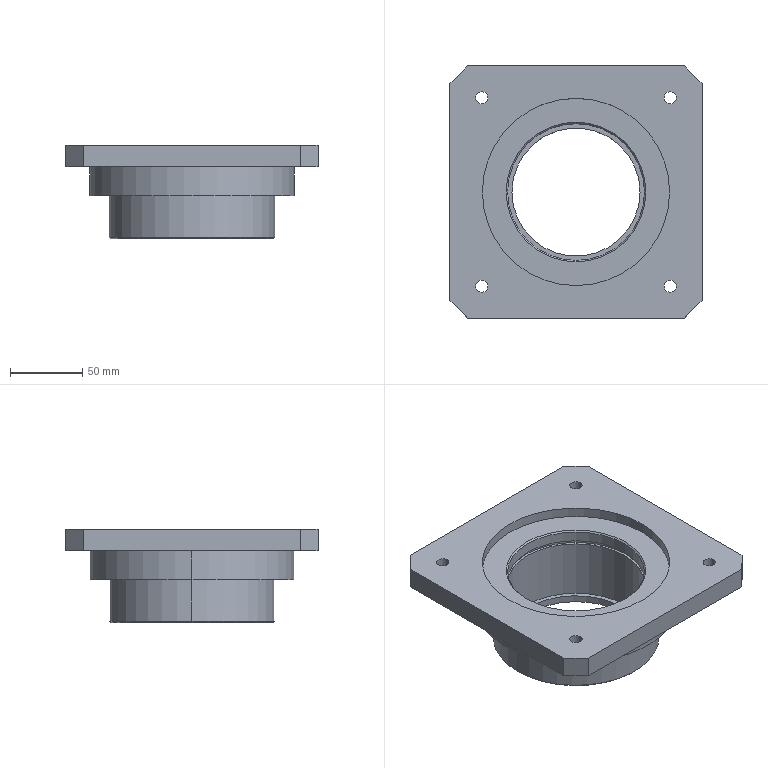Component | SolidWorks | PlanetaryReducer-PLF142BearingHousing-1 | 1 solid | 42 faces | box 175 x 175 x 65 mm | volume 578532 mm3 | cylinder 22 | plane 16 | cone 4 | commonest cylinder face diameters 8.5 x8 95 x4 130 x2 98.5 x2 142 x2 115 x2 89 x2
build123d program:
from build123d import *

# Parameters (mm, degrees)
SKETCH1_R           = 57.5
BOSS_EXTRUDE1_DEPTH = 30
SKETCH2_R           = 71
BOSS_EXTRUDE2_DEPTH = 20
SKETCH3_R           = 65
BOSS_EXTRUDE3_DEPTH = 8
SKETCH4_R           = 44.5
CUT_EXTRUDE1_DEPTH  = 116.957
SKETCH5_R           = 47.5
CUT_EXTRUDE2_DEPTH  = 53
CUT_EXTRUDE3_START  = -8.3
SKETCH6_R           = 49.25
CUT_EXTRUDE3_DEPTH  = 2.7
CHAMFER1_SIZE       = 1
SKETCH7_W           = 175
SKETCH7_H           = 175
SKETCH7_R           = 65
BOSS_EXTRUDE4_DEPTH = 15
CHAMFER2_SIZE       = 12
M10_TAPPED_HOLE1_D  = 8.5


with BuildPart() as part:
    # Sketch1 → Boss-Extrude1 (new body)
    with BuildSketch(Plane(origin=(0, 0, 0), x_dir=(1, 0, 0), z_dir=(0, 1, 0))):
        with Locations(Location((0, 0, 0), (0, 0, 270))):
            Circle(SKETCH1_R)
    extrude(amount=BOSS_EXTRUDE1_DEPTH)

    # Sketch2 → Boss-Extrude2 (add)
    with BuildSketch(Plane(origin=(0, 30, 0), x_dir=(1, 0, 0), z_dir=(0, 1, 0))):
        with Locations(Location((0, 0, 0), (0, 0, 270))):
            Circle(SKETCH2_R)
    extrude(amount=BOSS_EXTRUDE2_DEPTH)

    # Sketch3 → Boss-Extrude3 (add)
    with BuildSketch(Plane(origin=(0, 50, 0), x_dir=(1, 0, 0), z_dir=(0, 1, 0))):
        with Locations(Location((0, 0, 0), (0, 0, 270))):
            Circle(SKETCH3_R)
    extrude(amount=BOSS_EXTRUDE3_DEPTH)

    # Sketch4 → Cut-Extrude1 (cut, through all)
    with BuildSketch(Plane(origin=(0, 58, 0), x_dir=(1, 0, 0), z_dir=(0, 1, 0))):
        with Locations(Location((0, 0, 0), (0, 0, 270))):
            Circle(SKETCH4_R)
    extrude(amount=-CUT_EXTRUDE1_DEPTH, mode=Mode.SUBTRACT)

    # Sketch5 → Cut-Extrude2 (cut)
    with BuildSketch(Plane(origin=(0, 58, 0), x_dir=(1, 0, 0), z_dir=(0, 1, 0))):
        with Locations(Location((0, 0, 0), (0, 0, 270))):
            Circle(SKETCH5_R)
    extrude(amount=-CUT_EXTRUDE2_DEPTH, mode=Mode.SUBTRACT)

    # Sketch6 → Cut-Extrude3 (cut)
    with BuildSketch(Plane(origin=(0, 58, 0), x_dir=(1, 0, 0), z_dir=(0, 1, 0)).offset(CUT_EXTRUDE3_START)):
        with Locations(Location((0, 0, 0), (0, 0, 270))):
            Circle(SKETCH6_R)
    extrude(amount=-CUT_EXTRUDE3_DEPTH, mode=Mode.SUBTRACT)

    # Chamfer1
    chamfer1_edges = [part.edges().sort_by_distance(p)[0] for p in [
        (0, 0, -57.5),
        (0, 58, -47.5),
    ]]
    chamfer(chamfer1_edges, length=CHAMFER1_SIZE)

    # Sketch7 → Boss-Extrude4 (add)
    with BuildSketch(Plane(origin=(0, 50, 0), x_dir=(1, 0, 0), z_dir=(0, 1, 0))):
        Rectangle(SKETCH7_W, SKETCH7_H)
        with Locations(Location((0, 0, 0), (0, 0, 270))):
            Circle(SKETCH7_R, mode=Mode.SUBTRACT)
    extrude(amount=BOSS_EXTRUDE4_DEPTH)

    # Chamfer2
    chamfer2_edges = [part.edges().sort_by_distance(p)[0] for p in [
        (87.5, 57.5, 87.5),
        (87.5, 57.5, -87.5),
        (-87.5, 57.5, -87.5),
        (-87.5, 57.5, 87.5),
    ]]
    chamfer(chamfer2_edges, length=CHAMFER2_SIZE)

    # M10 Tapped Hole1 (through all)
    with Locations(Plane(origin=(-65.405, 65, -65.405), x_dir=(0, 0, 1), z_dir=(0, 1, 0))):
        with Locations((0, 0), (130.81, 0), (130.81, 130.81), (0, 130.81)):
            Hole(M10_TAPPED_HOLE1_D / 2)


solid = part.part

# Placed as in the assembly
solid = solid.moved(Location((-85, 178, 92), (90, 0, 0)))